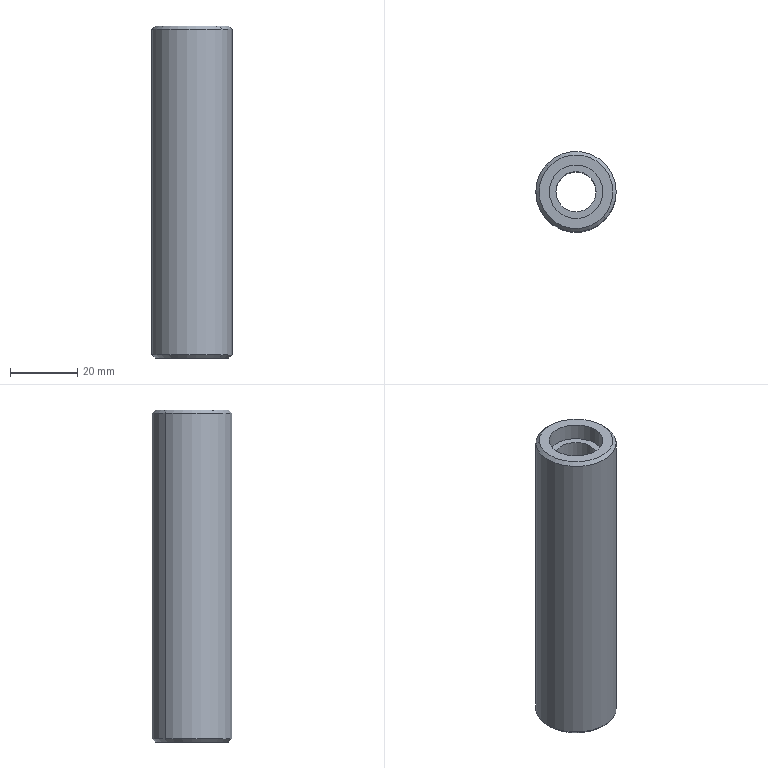Component | SolidWorks | TAR-02-023KnurledPaperPressWheel-1 | 1 solid | 16 faces | box 24 x 24 x 99 mm | volume 32637 mm3 | cylinder 8 | cone 4 | plane 4 | commonest cylinder face diameters 16 x4 24 x2 12 x2
build123d program:
from build123d import *

# Parameters (mm, degrees)
SKETCH1_R           = 12
SKETCH1_R_2         = 6
BOSS_EXTRUDE1_DEPTH = 99
CHAMFER1_SIZE       = 1
SKETCH2_R           = 8
CUT_EXTRUDE1_DEPTH  = 5
CUT_EXTRUDE2_START  = -5
SKETCH3_R           = 8
CUT_EXTRUDE2_DEPTH  = 5


with BuildPart() as part:
    # Sketch1 → Boss-Extrude1 (new body)
    with BuildSketch(Plane.XY):
        Circle(SKETCH1_R)
        Circle(SKETCH1_R_2, mode=Mode.SUBTRACT)
    extrude(amount=BOSS_EXTRUDE1_DEPTH)

    # Chamfer1
    chamfer1_edges = [part.edges().sort_by_distance(p)[0] for p in [
        (-12, 0, 0),
        (-12, 0, 99),
    ]]
    chamfer(chamfer1_edges, length=CHAMFER1_SIZE)

    # Sketch2 → Cut-Extrude1 (cut)
    with BuildSketch(Plane.XY.offset(99)):
        Circle(SKETCH2_R)
    extrude(amount=-CUT_EXTRUDE1_DEPTH, mode=Mode.SUBTRACT)

    # Sketch3 → Cut-Extrude2 (cut)
    with BuildSketch(Plane(origin=(0, 0, 0), x_dir=(-1, 0, 0), z_dir=(0, 0, -1)).offset(CUT_EXTRUDE2_START)):
        with Locations(Location((0, 0, 0), (0, 0, 180))):
            Circle(SKETCH3_R)
    extrude(amount=CUT_EXTRUDE2_DEPTH, mode=Mode.SUBTRACT)


solid = part.part

# Placed as in the assembly
solid = solid.moved(Location((8.333, 43.101, -143.165), (0, 0, 0)))
STEP:
#1=COLOUR_RGB('',0.7922,0.8196,0.9333);
#2=FILL_AREA_STYLE_COLOUR('',#1);
#3=FILL_AREA_STYLE('',(#2));
#4=SURFACE_STYLE_FILL_AREA(#3);
#5=SURFACE_SIDE_STYLE('',(#4));
#6=SURFACE_STYLE_USAGE(.BOTH.,#5);
#7=PRESENTATION_STYLE_ASSIGNMENT((#6));
#8=CARTESIAN_POINT('',(0.5621,1.486,-5.44));
#9=VERTEX_POINT('',#8);
#10=CARTESIAN_POINT('',(0.09403,1.908,-5.44));
#11=VERTEX_POINT('',#10);
#12=CARTESIAN_POINT('',(0.3281,1.697,-5.44));
#13=DIRECTION('',(0.,0.,-1.));
#14=DIRECTION('',(-0.743,0.6692,0.));
#15=AXIS2_PLACEMENT_3D('',#12,#13,#14);
#16=CIRCLE('',#15,0.315);
#17=EDGE_CURVE('',#9,#11,#16,.T.);
#18=ORIENTED_EDGE('',*,*,#17,.F.);
#19=CARTESIAN_POINT('',(0.5621,1.486,-5.636));
#20=VERTEX_POINT('',#19);
#21=CARTESIAN_POINT('',(0.5621,1.486,-5.44));
#22=DIRECTION('',(0.,0.,-1.));
#23=VECTOR('',#22,39.37);
#24=LINE('',#21,#23);
#25=EDGE_CURVE('',#9,#20,#24,.T.);
#26=ORIENTED_EDGE('',*,*,#25,.T.);
#27=CARTESIAN_POINT('',(0.09403,1.908,-5.636));
#28=VERTEX_POINT('',#27);
#29=CARTESIAN_POINT('',(0.3281,1.697,-5.636));
#30=DIRECTION('',(0.,0.,-1.));
#31=DIRECTION('',(-0.743,0.6692,0.));
#32=AXIS2_PLACEMENT_3D('',#29,#30,#31);
#33=CIRCLE('',#32,0.315);
#34=EDGE_CURVE('',#20,#28,#33,.T.);
#35=ORIENTED_EDGE('',*,*,#34,.T.);
#36=CARTESIAN_POINT('',(0.09403,1.908,-5.44));
#37=DIRECTION('',(0.,0.,-1.));
#38=VECTOR('',#37,39.37);
#39=LINE('',#36,#38);
#40=EDGE_CURVE('',#11,#28,#39,.T.);
#41=ORIENTED_EDGE('',*,*,#40,.F.);
#42=EDGE_LOOP('',(#18,#26,#35,#41));
#43=FACE_OUTER_BOUND('',#42,.T.);
#44=CARTESIAN_POINT('',(0.3281,1.697,-5.44));
#45=DIRECTION('',(0.,0.,-1.));
#46=DIRECTION('',(-0.743,0.6692,0.));
#47=AXIS2_PLACEMENT_3D('',#44,#45,#46);
#48=CYLINDRICAL_SURFACE('',#47,0.315);
#49=ADVANCED_FACE('',(#43),#48,.F.);
#50=CARTESIAN_POINT('',(0.09403,1.908,-1.936));
#51=VERTEX_POINT('',#50);
#52=CARTESIAN_POINT('',(0.5621,1.486,-1.936));
#53=VERTEX_POINT('',#52);
#54=CARTESIAN_POINT('',(0.3281,1.697,-1.936));
#55=DIRECTION('',(0.,0.,1.));
#56=DIRECTION('',(0.743,-0.6692,0.));
#57=AXIS2_PLACEMENT_3D('',#54,#55,#56);
#58=CIRCLE('',#57,0.315);
#59=EDGE_CURVE('',#51,#53,#58,.T.);
#60=ORIENTED_EDGE('',*,*,#59,.F.);
#61=CARTESIAN_POINT('',(0.09403,1.908,-1.739));
#62=VERTEX_POINT('',#61);
#63=CARTESIAN_POINT('',(0.09403,1.908,-1.936));
#64=DIRECTION('',(0.,0.,1.));
#65=VECTOR('',#64,39.37);
#66=LINE('',#63,#65);
#67=EDGE_CURVE('',#51,#62,#66,.T.);
#68=ORIENTED_EDGE('',*,*,#67,.T.);
#69=CARTESIAN_POINT('',(0.5621,1.486,-1.739));
#70=VERTEX_POINT('',#69);
#71=CARTESIAN_POINT('',(0.3281,1.697,-1.739));
#72=DIRECTION('',(0.,0.,1.));
#73=DIRECTION('',(0.743,-0.6692,0.));
#74=AXIS2_PLACEMENT_3D('',#71,#72,#73);
#75=CIRCLE('',#74,0.315);
#76=EDGE_CURVE('',#62,#70,#75,.T.);
#77=ORIENTED_EDGE('',*,*,#76,.T.);
#78=CARTESIAN_POINT('',(0.5621,1.486,-1.936));
#79=DIRECTION('',(0.,0.,1.));
#80=VECTOR('',#79,39.37);
#81=LINE('',#78,#80);
#82=EDGE_CURVE('',#53,#70,#81,.T.);
#83=ORIENTED_EDGE('',*,*,#82,.F.);
#84=EDGE_LOOP('',(#60,#68,#77,#83));
#85=FACE_OUTER_BOUND('',#84,.T.);
#86=CARTESIAN_POINT('',(0.3281,1.697,-1.936));
#87=DIRECTION('',(0.,0.,1.));
#88=DIRECTION('',(0.743,-0.6692,0.));
#89=AXIS2_PLACEMENT_3D('',#86,#87,#88);
#90=CYLINDRICAL_SURFACE('',#89,0.315);
#91=ADVANCED_FACE('',(#85),#90,.F.);
#92=CARTESIAN_POINT('',(0.6498,1.407,-1.739));
#93=VERTEX_POINT('',#92);
#94=CARTESIAN_POINT('',(0.00627,1.987,-1.739));
#95=VERTEX_POINT('',#94);
#96=CARTESIAN_POINT('',(0.3281,1.697,-1.739));
#97=DIRECTION('',(0.,0.,1.));
#98=DIRECTION('',(0.743,-0.6692,0.));
#99=AXIS2_PLACEMENT_3D('',#96,#97,#98);
#100=CIRCLE('',#99,0.4331);
#101=EDGE_CURVE('',#93,#95,#100,.T.);
#102=ORIENTED_EDGE('',*,*,#101,.F.);
#103=CARTESIAN_POINT('',(0.6791,1.381,-1.778));
#104=VERTEX_POINT('',#103);
#105=CARTESIAN_POINT('',(0.6498,1.407,-1.739));
#106=DIRECTION('',(0.5254,-0.4732,-0.7071));
#107=VECTOR('',#106,39.37);
#108=LINE('',#105,#107);
#109=EDGE_CURVE('',#93,#104,#108,.T.);
#110=ORIENTED_EDGE('',*,*,#109,.T.);
#111=CARTESIAN_POINT('',(-0.02298,2.013,-1.778));
#112=VERTEX_POINT('',#111);
#113=CARTESIAN_POINT('',(0.3281,1.697,-1.778));
#114=DIRECTION('',(0.,0.,-1.));
#115=DIRECTION('',(0.743,-0.6692,0.));
#116=AXIS2_PLACEMENT_3D('',#113,#114,#115);
#117=CIRCLE('',#116,0.4724);
#118=EDGE_CURVE('',#112,#104,#117,.T.);
#119=ORIENTED_EDGE('',*,*,#118,.F.);
#120=CARTESIAN_POINT('',(0.00627,1.987,-1.739));
#121=DIRECTION('',(-0.5254,0.4732,-0.7071));
#122=VECTOR('',#121,39.37);
#123=LINE('',#120,#122);
#124=EDGE_CURVE('',#95,#112,#123,.T.);
#125=ORIENTED_EDGE('',*,*,#124,.F.);
#126=EDGE_LOOP('',(#102,#110,#119,#125));
#127=FACE_OUTER_BOUND('',#126,.T.);
#128=CARTESIAN_POINT('',(0.3281,1.697,-1.739));
#129=DIRECTION('',(0.,0.,-1.));
#130=DIRECTION('',(-0.743,0.6692,0.));
#131=AXIS2_PLACEMENT_3D('',#128,#129,#130);
#132=CONICAL_SURFACE('',#131,0.4331,0.7854);
#133=ADVANCED_FACE('',(#127),#132,.T.);
#134=CARTESIAN_POINT('',(0.00627,1.987,-5.636));
#135=VERTEX_POINT('',#134);
#136=CARTESIAN_POINT('',(0.6498,1.407,-5.636));
#137=VERTEX_POINT('',#136);
#138=CARTESIAN_POINT('',(0.3281,1.697,-5.636));
#139=DIRECTION('',(0.,0.,-1.));
#140=DIRECTION('',(0.743,-0.6692,0.));
#141=AXIS2_PLACEMENT_3D('',#138,#139,#140);
#142=CIRCLE('',#141,0.4331);
#143=EDGE_CURVE('',#135,#137,#142,.T.);
#144=ORIENTED_EDGE('',*,*,#143,.F.);
#145=CARTESIAN_POINT('',(-0.02298,2.013,-5.597));
#146=VERTEX_POINT('',#145);
#147=CARTESIAN_POINT('',(-0.02298,2.013,-5.597));
#148=DIRECTION('',(-0.5254,0.4732,0.7071));
#149=VECTOR('',#148,39.37);
#150=LINE('',#147,#149);
#151=EDGE_CURVE('',#135,#146,#150,.T.);
#152=ORIENTED_EDGE('',*,*,#151,.T.);
#153=CARTESIAN_POINT('',(0.6791,1.381,-5.597));
#154=VERTEX_POINT('',#153);
#155=CARTESIAN_POINT('',(0.3281,1.697,-5.597));
#156=DIRECTION('',(0.,0.,1.));
#157=DIRECTION('',(0.743,-0.6692,0.));
#158=AXIS2_PLACEMENT_3D('',#155,#156,#157);
#159=CIRCLE('',#158,0.4724);
#160=EDGE_CURVE('',#154,#146,#159,.T.);
#161=ORIENTED_EDGE('',*,*,#160,.F.);
#162=CARTESIAN_POINT('',(0.6791,1.381,-5.597));
#163=DIRECTION('',(0.5254,-0.4732,0.7071));
#164=VECTOR('',#163,39.37);
#165=LINE('',#162,#164);
#166=EDGE_CURVE('',#137,#154,#165,.T.);
#167=ORIENTED_EDGE('',*,*,#166,.F.);
#168=EDGE_LOOP('',(#144,#152,#161,#167));
#169=FACE_OUTER_BOUND('',#168,.T.);
#170=CARTESIAN_POINT('',(0.3281,1.697,-5.597));
#171=DIRECTION('',(0.,0.,1.));
#172=DIRECTION('',(0.743,-0.6692,0.));
#173=AXIS2_PLACEMENT_3D('',#170,#171,#172);
#174=CONICAL_SURFACE('',#173,0.4724,0.7854);
#175=ADVANCED_FACE('',(#169),#174,.T.);
#176=ORIENTED_EDGE('',*,*,#118,.T.);
#177=CARTESIAN_POINT('',(0.6791,1.381,-1.739));
#178=DIRECTION('',(0.,0.,-1.));
#179=VECTOR('',#178,39.37);
#180=LINE('',#177,#179);
#181=EDGE_CURVE('',#104,#154,#180,.T.);
#182=ORIENTED_EDGE('',*,*,#181,.T.);
#183=ORIENTED_EDGE('',*,*,#160,.T.);
#184=CARTESIAN_POINT('',(-0.02298,2.013,-1.739));
#185=DIRECTION('',(0.,0.,-1.));
#186=VECTOR('',#185,39.37);
#187=LINE('',#184,#186);
#188=EDGE_CURVE('',#112,#146,#187,.T.);
#189=ORIENTED_EDGE('',*,*,#188,.F.);
#190=EDGE_LOOP('',(#176,#182,#183,#189));
#191=FACE_OUTER_BOUND('',#190,.T.);
#192=CARTESIAN_POINT('',(0.3281,1.697,-1.739));
#193=DIRECTION('',(0.,0.,-1.));
#194=DIRECTION('',(-0.743,0.6692,0.));
#195=AXIS2_PLACEMENT_3D('',#192,#193,#194);
#196=CYLINDRICAL_SURFACE('',#195,0.4724);
#197=ADVANCED_FACE('',(#191),#196,.T.);
#198=CARTESIAN_POINT('',(0.1525,1.855,-1.936));
#199=VERTEX_POINT('',#198);
#200=CARTESIAN_POINT('',(0.5036,1.539,-1.936));
#201=VERTEX_POINT('',#200);
#202=CARTESIAN_POINT('',(0.3281,1.697,-1.936));
#203=DIRECTION('',(0.,0.,1.));
#204=DIRECTION('',(0.743,-0.6692,0.));
#205=AXIS2_PLACEMENT_3D('',#202,#203,#204);
#206=CIRCLE('',#205,0.2362);
#207=EDGE_CURVE('',#199,#201,#206,.T.);
#208=ORIENTED_EDGE('',*,*,#207,.T.);
#209=CARTESIAN_POINT('',(0.5036,1.539,-5.44));
#210=VERTEX_POINT('',#209);
#211=CARTESIAN_POINT('',(0.5036,1.539,-1.739));
#212=DIRECTION('',(0.,0.,-1.));
#213=VECTOR('',#212,39.37);
#214=LINE('',#211,#213);
#215=EDGE_CURVE('',#201,#210,#214,.T.);
#216=ORIENTED_EDGE('',*,*,#215,.T.);
#217=CARTESIAN_POINT('',(0.1525,1.855,-5.44));
#218=VERTEX_POINT('',#217);
#219=CARTESIAN_POINT('',(0.3281,1.697,-5.44));
#220=DIRECTION('',(0.,0.,-1.));
#221=DIRECTION('',(-0.743,0.6692,0.));
#222=AXIS2_PLACEMENT_3D('',#219,#220,#221);
#223=CIRCLE('',#222,0.2362);
#224=EDGE_CURVE('',#210,#218,#223,.T.);
#225=ORIENTED_EDGE('',*,*,#224,.T.);
#226=CARTESIAN_POINT('',(0.1525,1.855,-1.739));
#227=DIRECTION('',(0.,0.,-1.));
#228=VECTOR('',#227,39.37);
#229=LINE('',#226,#228);
#230=EDGE_CURVE('',#199,#218,#229,.T.);
#231=ORIENTED_EDGE('',*,*,#230,.F.);
#232=EDGE_LOOP('',(#208,#216,#225,#231));
#233=FACE_OUTER_BOUND('',#232,.T.);
#234=CARTESIAN_POINT('',(0.3281,1.697,-1.739));
#235=DIRECTION('',(0.,0.,-1.));
#236=DIRECTION('',(-0.743,0.6692,0.));
#237=AXIS2_PLACEMENT_3D('',#234,#235,#236);
#238=CYLINDRICAL_SURFACE('',#237,0.2362);
#239=ADVANCED_FACE('',(#233),#238,.F.);
#240=ORIENTED_EDGE('',*,*,#215,.F.);
#241=CARTESIAN_POINT('',(0.3281,1.697,-1.936));
#242=DIRECTION('',(0.,0.,1.));
#243=DIRECTION('',(0.743,-0.6692,0.));
#244=AXIS2_PLACEMENT_3D('',#241,#242,#243);
#245=CIRCLE('',#244,0.2362);
#246=EDGE_CURVE('',#201,#199,#245,.T.);
#247=ORIENTED_EDGE('',*,*,#246,.T.);
#248=ORIENTED_EDGE('',*,*,#230,.T.);
#249=CARTESIAN_POINT('',(0.3281,1.697,-5.44));
#250=DIRECTION('',(0.,0.,-1.));
#251=DIRECTION('',(-0.743,0.6692,0.));
#252=AXIS2_PLACEMENT_3D('',#249,#250,#251);
#253=CIRCLE('',#252,0.2362);
#254=EDGE_CURVE('',#218,#210,#253,.T.);
#255=ORIENTED_EDGE('',*,*,#254,.T.);
#256=EDGE_LOOP('',(#240,#247,#248,#255));
#257=FACE_OUTER_BOUND('',#256,.T.);
#258=CARTESIAN_POINT('',(0.3281,1.697,-1.739));
#259=DIRECTION('',(0.,0.,-1.));
#260=DIRECTION('',(-0.743,0.6692,0.));
#261=AXIS2_PLACEMENT_3D('',#258,#259,#260);
#262=CYLINDRICAL_SURFACE('',#261,0.2362);
#263=ADVANCED_FACE('',(#257),#262,.F.);
#264=CARTESIAN_POINT('',(0.3281,1.697,-1.739));
#265=DIRECTION('',(0.,0.,1.));
#266=DIRECTION('',(0.743,-0.6692,0.));
#267=AXIS2_PLACEMENT_3D('',#264,#265,#266);
#268=CIRCLE('',#267,0.315);
#269=EDGE_CURVE('',#70,#62,#268,.T.);
#270=ORIENTED_EDGE('',*,*,#269,.F.);
#271=ORIENTED_EDGE('',*,*,#76,.F.);
#272=EDGE_LOOP('',(#270,#271));
#273=FACE_BOUND('',#272,.T.);
#274=CARTESIAN_POINT('',(0.3281,1.697,-1.739));
#275=DIRECTION('',(0.,0.,1.));
#276=DIRECTION('',(0.743,-0.6692,0.));
#277=AXIS2_PLACEMENT_3D('',#274,#275,#276);
#278=CIRCLE('',#277,0.4331);
#279=EDGE_CURVE('',#95,#93,#278,.T.);
#280=ORIENTED_EDGE('',*,*,#279,.T.);
#281=ORIENTED_EDGE('',*,*,#101,.T.);
#282=EDGE_LOOP('',(#280,#281));
#283=FACE_OUTER_BOUND('',#282,.T.);
#284=CARTESIAN_POINT('',(0.3281,1.697,-1.739));
#285=DIRECTION('',(0.,0.,1.));
#286=DIRECTION('',(0.743,-0.6692,0.));
#287=AXIS2_PLACEMENT_3D('',#284,#285,#286);
#288=PLANE('',#287);
#289=ADVANCED_FACE('',(#273,#283),#288,.T.);
#290=CARTESIAN_POINT('',(0.3281,1.697,-5.636));
#291=DIRECTION('',(0.,0.,-1.));
#292=DIRECTION('',(-0.743,0.6692,0.));
#293=AXIS2_PLACEMENT_3D('',#290,#291,#292);
#294=CIRCLE('',#293,0.315);
#295=EDGE_CURVE('',#28,#20,#294,.T.);
#296=ORIENTED_EDGE('',*,*,#295,.F.);
#297=ORIENTED_EDGE('',*,*,#34,.F.);
#298=EDGE_LOOP('',(#296,#297));
#299=FACE_BOUND('',#298,.T.);
#300=CARTESIAN_POINT('',(0.3281,1.697,-5.636));
#301=DIRECTION('',(0.,0.,-1.));
#302=DIRECTION('',(0.743,-0.6692,0.));
#303=AXIS2_PLACEMENT_3D('',#300,#301,#302);
#304=CIRCLE('',#303,0.4331);
#305=EDGE_CURVE('',#137,#135,#304,.T.);
#306=ORIENTED_EDGE('',*,*,#305,.T.);
#307=ORIENTED_EDGE('',*,*,#143,.T.);
#308=EDGE_LOOP('',(#306,#307));
#309=FACE_OUTER_BOUND('',#308,.T.);
#310=CARTESIAN_POINT('',(0.3281,1.697,-5.636));
#311=DIRECTION('',(0.,0.,1.));
#312=DIRECTION('',(0.743,-0.6692,0.));
#313=AXIS2_PLACEMENT_3D('',#310,#311,#312);
#314=PLANE('',#313);
#315=ADVANCED_FACE('',(#299,#309),#314,.F.);
#316=ORIENTED_EDGE('',*,*,#181,.F.);
#317=CARTESIAN_POINT('',(0.3281,1.697,-1.778));
#318=DIRECTION('',(0.,0.,-1.));
#319=DIRECTION('',(0.743,-0.6692,0.));
#320=AXIS2_PLACEMENT_3D('',#317,#318,#319);
#321=CIRCLE('',#320,0.4724);
#322=EDGE_CURVE('',#104,#112,#321,.T.);
#323=ORIENTED_EDGE('',*,*,#322,.T.);
#324=ORIENTED_EDGE('',*,*,#188,.T.);
#325=CARTESIAN_POINT('',(0.3281,1.697,-5.597));
#326=DIRECTION('',(0.,0.,1.));
#327=DIRECTION('',(0.743,-0.6692,0.));
#328=AXIS2_PLACEMENT_3D('',#325,#326,#327);
#329=CIRCLE('',#328,0.4724);
#330=EDGE_CURVE('',#146,#154,#329,.T.);
#331=ORIENTED_EDGE('',*,*,#330,.T.);
#332=EDGE_LOOP('',(#316,#323,#324,#331));
#333=FACE_OUTER_BOUND('',#332,.T.);
#334=CARTESIAN_POINT('',(0.3281,1.697,-1.739));
#335=DIRECTION('',(0.,0.,-1.));
#336=DIRECTION('',(-0.743,0.6692,0.));
#337=AXIS2_PLACEMENT_3D('',#334,#335,#336);
#338=CYLINDRICAL_SURFACE('',#337,0.4724);
#339=ADVANCED_FACE('',(#333),#338,.T.);
#340=ORIENTED_EDGE('',*,*,#151,.F.);
#341=ORIENTED_EDGE('',*,*,#305,.F.);
#342=ORIENTED_EDGE('',*,*,#166,.T.);
#343=ORIENTED_EDGE('',*,*,#330,.F.);
#344=EDGE_LOOP('',(#340,#341,#342,#343));
#345=FACE_OUTER_BOUND('',#344,.T.);
#346=CARTESIAN_POINT('',(0.3281,1.697,-5.597));
#347=DIRECTION('',(0.,0.,1.));
#348=DIRECTION('',(0.743,-0.6692,0.));
#349=AXIS2_PLACEMENT_3D('',#346,#347,#348);
#350=CONICAL_SURFACE('',#349,0.4724,0.7854);
#351=ADVANCED_FACE('',(#345),#350,.T.);
#352=ORIENTED_EDGE('',*,*,#109,.F.);
#353=ORIENTED_EDGE('',*,*,#279,.F.);
#354=ORIENTED_EDGE('',*,*,#124,.T.);
#355=ORIENTED_EDGE('',*,*,#322,.F.);
#356=EDGE_LOOP('',(#352,#353,#354,#355));
#357=FACE_OUTER_BOUND('',#356,.T.);
#358=CARTESIAN_POINT('',(0.3281,1.697,-1.739));
#359=DIRECTION('',(0.,0.,-1.));
#360=DIRECTION('',(-0.743,0.6692,0.));
#361=AXIS2_PLACEMENT_3D('',#358,#359,#360);
#362=CONICAL_SURFACE('',#361,0.4331,0.7854);
#363=ADVANCED_FACE('',(#357),#362,.T.);
#364=ORIENTED_EDGE('',*,*,#67,.F.);
#365=CARTESIAN_POINT('',(0.3281,1.697,-1.936));
#366=DIRECTION('',(0.,0.,1.));
#367=DIRECTION('',(0.743,-0.6692,0.));
#368=AXIS2_PLACEMENT_3D('',#365,#366,#367);
#369=CIRCLE('',#368,0.315);
#370=EDGE_CURVE('',#53,#51,#369,.T.);
#371=ORIENTED_EDGE('',*,*,#370,.F.);
#372=ORIENTED_EDGE('',*,*,#82,.T.);
#373=ORIENTED_EDGE('',*,*,#269,.T.);
#374=EDGE_LOOP('',(#364,#371,#372,#373));
#375=FACE_OUTER_BOUND('',#374,.T.);
#376=CARTESIAN_POINT('',(0.3281,1.697,-1.936));
#377=DIRECTION('',(0.,0.,1.));
#378=DIRECTION('',(0.743,-0.6692,0.));
#379=AXIS2_PLACEMENT_3D('',#376,#377,#378);
#380=CYLINDRICAL_SURFACE('',#379,0.315);
#381=ADVANCED_FACE('',(#375),#380,.F.);
#382=ORIENTED_EDGE('',*,*,#207,.F.);
#383=ORIENTED_EDGE('',*,*,#246,.F.);
#384=EDGE_LOOP('',(#382,#383));
#385=FACE_BOUND('',#384,.T.);
#386=ORIENTED_EDGE('',*,*,#370,.T.);
#387=ORIENTED_EDGE('',*,*,#59,.T.);
#388=EDGE_LOOP('',(#386,#387));
#389=FACE_OUTER_BOUND('',#388,.T.);
#390=CARTESIAN_POINT('',(0.3281,1.697,-1.936));
#391=DIRECTION('',(0.,0.,1.));
#392=DIRECTION('',(0.743,-0.6692,0.));
#393=AXIS2_PLACEMENT_3D('',#390,#391,#392);
#394=PLANE('',#393);
#395=ADVANCED_FACE('',(#385,#389),#394,.T.);
#396=ORIENTED_EDGE('',*,*,#25,.F.);
#397=CARTESIAN_POINT('',(0.3281,1.697,-5.44));
#398=DIRECTION('',(0.,0.,-1.));
#399=DIRECTION('',(-0.743,0.6692,0.));
#400=AXIS2_PLACEMENT_3D('',#397,#398,#399);
#401=CIRCLE('',#400,0.315);
#402=EDGE_CURVE('',#11,#9,#401,.T.);
#403=ORIENTED_EDGE('',*,*,#402,.F.);
#404=ORIENTED_EDGE('',*,*,#40,.T.);
#405=ORIENTED_EDGE('',*,*,#295,.T.);
#406=EDGE_LOOP('',(#396,#403,#404,#405));
#407=FACE_OUTER_BOUND('',#406,.T.);
#408=CARTESIAN_POINT('',(0.3281,1.697,-5.44));
#409=DIRECTION('',(0.,0.,-1.));
#410=DIRECTION('',(-0.743,0.6692,0.));
#411=AXIS2_PLACEMENT_3D('',#408,#409,#410);
#412=CYLINDRICAL_SURFACE('',#411,0.315);
#413=ADVANCED_FACE('',(#407),#412,.F.);
#414=ORIENTED_EDGE('',*,*,#254,.F.);
#415=ORIENTED_EDGE('',*,*,#224,.F.);
#416=EDGE_LOOP('',(#414,#415));
#417=FACE_BOUND('',#416,.T.);
#418=ORIENTED_EDGE('',*,*,#402,.T.);
#419=ORIENTED_EDGE('',*,*,#17,.T.);
#420=EDGE_LOOP('',(#418,#419));
#421=FACE_OUTER_BOUND('',#420,.T.);
#422=CARTESIAN_POINT('',(0.3281,1.697,-5.44));
#423=DIRECTION('',(0.,0.,-1.));
#424=DIRECTION('',(-0.743,0.6692,0.));
#425=AXIS2_PLACEMENT_3D('',#422,#423,#424);
#426=PLANE('',#425);
#427=ADVANCED_FACE('',(#417,#421),#426,.T.);
#428=CLOSED_SHELL('',(#49,#91,#133,#175,#197,#239,#263,#289,#315,#339,#351,#363,#381,#395,#413,#427));
#429=MANIFOLD_SOLID_BREP('',#428);
#430=STYLED_ITEM('',(#7),#429);
#431=PRESENTATION_LAYER_ASSIGNMENT('','',(#430));
#432=CARTESIAN_POINT('',(0.,0.,0.));
#433=DIRECTION('',(0.,0.,1.));
#434=DIRECTION('',(1.,0.,0.));
#435=AXIS2_PLACEMENT_3D('',#432,#433,#434);
#436=(LENGTH_UNIT()NAMED_UNIT(*)SI_UNIT($,.METRE.));
#437=LENGTH_MEASURE_WITH_UNIT(LENGTH_MEASURE(0.0254),#436);
#438=DIMENSIONAL_EXPONENTS(1.,0.,0.,0.,0.,0.,0.);
#439=(CONVERSION_BASED_UNIT('',#437)LENGTH_UNIT()NAMED_UNIT(#438));
#440=UNCERTAINTY_MEASURE_WITH_UNIT(LENGTH_MEASURE(0.00001),#439,'','');
#441=(NAMED_UNIT(*)PLANE_ANGLE_UNIT()SI_UNIT($,.RADIAN.));
#442=(NAMED_UNIT(*)SI_UNIT($,.STERADIAN.)SOLID_ANGLE_UNIT());
#443=(GEOMETRIC_REPRESENTATION_CONTEXT(3)GLOBAL_UNCERTAINTY_ASSIGNED_CONTEXT((#440))GLOBAL_UNIT_ASSIGNED_CONTEXT((#439,#441,#442))REPRESENTATION_CONTEXT('',''));
#444=ADVANCED_BREP_SHAPE_REPRESENTATION('',(#429,#435),#443);
#445=(LENGTH_UNIT()NAMED_UNIT(*)SI_UNIT($,.METRE.));
#446=LENGTH_MEASURE_WITH_UNIT(LENGTH_MEASURE(0.0254),#445);
#447=DIMENSIONAL_EXPONENTS(1.,0.,0.,0.,0.,0.,0.);
#448=(CONVERSION_BASED_UNIT('',#446)LENGTH_UNIT()NAMED_UNIT(#447));
#449=UNCERTAINTY_MEASURE_WITH_UNIT(LENGTH_MEASURE(0.00001),#448,'','');
#450=(NAMED_UNIT(*)PLANE_ANGLE_UNIT()SI_UNIT($,.RADIAN.));
#451=(NAMED_UNIT(*)SI_UNIT($,.STERADIAN.)SOLID_ANGLE_UNIT());
#452=(GEOMETRIC_REPRESENTATION_CONTEXT(3)GLOBAL_UNCERTAINTY_ASSIGNED_CONTEXT((#449))GLOBAL_UNIT_ASSIGNED_CONTEXT((#448,#450,#451))REPRESENTATION_CONTEXT('',''));
#453=MECHANICAL_DESIGN_GEOMETRIC_PRESENTATION_REPRESENTATION('',(#430),#452);